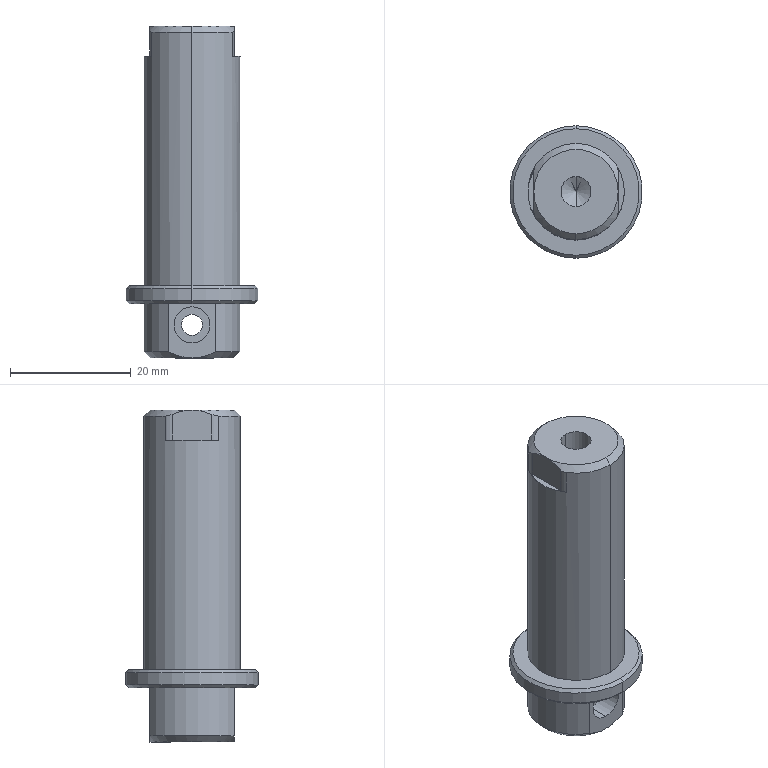Component | SolidWorks | DZ.KX.203-TC1505-30-09-01-05-22-2 | 1 solid | 41 faces | volume 10688 mm3 | cylinder 18 | plane 12 | cone 11 | commonest cylinder face diameters 16 x4 4 x4 6 x2 6.5 x2 3.5 x2 22 x2 5 x2 | material Cast Carbon Steel